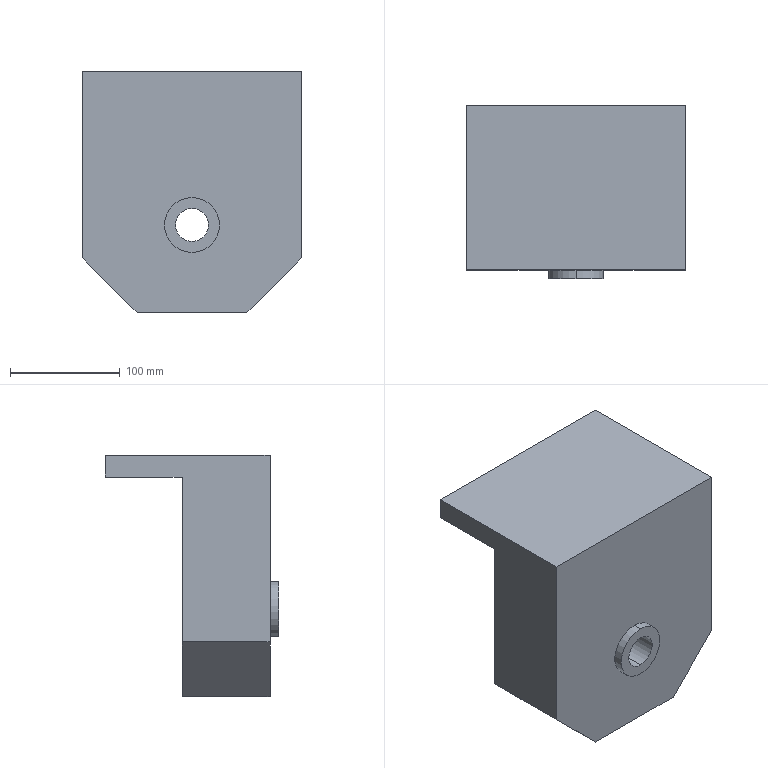Component | SolidWorks | HZ022-A001-D001-1 | 1 solid | 21 faces | box 200 x 158 x 220 mm | volume 3538459 mm3 | plane 13 | cylinder 8 | commonest cylinder face diameters 50 x4 16 x2 30 x2 | material AL6061
build123d program:
from build123d import *

# Parameters (mm, degrees)
SKETCH1_2_W               = 200
SKETCH1_2_H               = 220
BOSS_EXTRUDE1_DEPTH       = 150
SKETCH2_W                 = 200
SKETCH2_H                 = 200
CUT_EXTRUDE1_DEPTH        = 70
SKETCH3_R                 = 25
CUT_EXTRUDE2_DEPTH        = 5
SKETCH4_R                 = 25
BOSS_EXTRUDE2_DEPTH       = 8
SKETCH5_R                 = 15
CUT_EXTRUDE3_DEPTH        = 217.942
CHAMFER1_SIZE             = 50
SKETCH1_R                 = 8
MOTORSHAFTCLEARANCE_DEPTH = 26


with BuildPart() as part:
    # Sketch1_2 → Boss-Extrude1 (new body)
    with BuildSketch(Plane(origin=(0, 0, 0), x_dir=(1, 0, 0), z_dir=(0, 1, 0))):
        Rectangle(SKETCH1_2_W, SKETCH1_2_H)
    extrude(amount=BOSS_EXTRUDE1_DEPTH)

    # Sketch2 → Cut-Extrude1 (cut)
    with BuildSketch(Plane(origin=(0, 150, 0), x_dir=(1, 0, 0), z_dir=(0, 1, 0))):
        with Locations((0, 10)):
            Rectangle(SKETCH2_W, SKETCH2_H)
    extrude(amount=-CUT_EXTRUDE1_DEPTH, mode=Mode.SUBTRACT)

    # Sketch3 → Cut-Extrude2 (cut)
    with BuildSketch(Plane(origin=(0, 80, 0), x_dir=(1, 0, 0), z_dir=(0, 1, 0))):
        with Locations(Location((0, -50, 0), (0, 0, 270))):
            Circle(SKETCH3_R)
    extrude(amount=-CUT_EXTRUDE2_DEPTH, mode=Mode.SUBTRACT)

    # Sketch4 → Boss-Extrude2 (add)
    with BuildSketch(Plane.XZ):
        with Locations(Location((0, -30, 0), (0, 0, 90))):
            Circle(SKETCH4_R)
    extrude(amount=BOSS_EXTRUDE2_DEPTH)

    # Sketch5 → Cut-Extrude3 (cut, through all)
    with BuildSketch(Plane.XZ.offset(8)):
        with Locations(Location((0, -30, 0), (0, 0, 270))):
            Circle(SKETCH5_R)
    extrude(amount=-CUT_EXTRUDE3_DEPTH, mode=Mode.SUBTRACT)

    # Chamfer1
    chamfer1_edges = [part.edges().sort_by_distance(p)[0] for p in [
        (-100, 40, -110),
        (100, 40, -110),
    ]]
    chamfer(chamfer1_edges, length=CHAMFER1_SIZE)

    # Sketch1 → MotorShaftClearance (cut)
    with BuildSketch(Plane(origin=(0, 75, 0), x_dir=(1, 0, 0), z_dir=(0, 1, 0))):
        with Locations(Location((0, -50, 0), (0, 0, 270))):
            Circle(SKETCH1_R)
    extrude(amount=-MOTORSHAFTCLEARANCE_DEPTH, mode=Mode.SUBTRACT)


solid = part.part

# Placed as in the assembly
solid = solid.moved(Location((-12.865, -151.602, 510), (0, 0, 0)))
STEP:
#1=COLOUR_RGB('',0.7922,0.8196,0.9333);
#2=FILL_AREA_STYLE_COLOUR('',#1);
#3=FILL_AREA_STYLE('',(#2));
#4=SURFACE_STYLE_FILL_AREA(#3);
#5=SURFACE_SIDE_STYLE('',(#4));
#6=SURFACE_STYLE_USAGE(.BOTH.,#5);
#7=PRESENTATION_STYLE_ASSIGNMENT((#6));
#8=CARTESIAN_POINT('',(-0.5065,-4.039,21.732));
#9=VERTEX_POINT('',#8);
#10=CARTESIAN_POINT('',(-0.5065,-4.039,22.362));
#11=VERTEX_POINT('',#10);
#12=CARTESIAN_POINT('',(-0.5065,-4.039,22.047));
#13=DIRECTION('',(0.,1.,0.));
#14=DIRECTION('',(0.,0.,1.));
#15=AXIS2_PLACEMENT_3D('',#12,#13,#14);
#16=CIRCLE('',#15,0.315);
#17=EDGE_CURVE('',#9,#11,#16,.T.);
#18=ORIENTED_EDGE('',*,*,#17,.F.);
#19=CARTESIAN_POINT('',(-0.5065,-3.016,21.732));
#20=VERTEX_POINT('',#19);
#21=CARTESIAN_POINT('',(-0.5065,-4.039,21.732));
#22=DIRECTION('',(0.,1.,0.));
#23=VECTOR('',#22,39.37);
#24=LINE('',#21,#23);
#25=EDGE_CURVE('',#9,#20,#24,.T.);
#26=ORIENTED_EDGE('',*,*,#25,.T.);
#27=CARTESIAN_POINT('',(-0.5065,-3.016,22.362));
#28=VERTEX_POINT('',#27);
#29=CARTESIAN_POINT('',(-0.5065,-3.016,22.047));
#30=DIRECTION('',(0.,1.,0.));
#31=DIRECTION('',(0.,0.,1.));
#32=AXIS2_PLACEMENT_3D('',#29,#30,#31);
#33=CIRCLE('',#32,0.315);
#34=EDGE_CURVE('',#20,#28,#33,.T.);
#35=ORIENTED_EDGE('',*,*,#34,.T.);
#36=CARTESIAN_POINT('',(-0.5065,-4.039,22.362));
#37=DIRECTION('',(0.,1.,0.));
#38=VECTOR('',#37,39.37);
#39=LINE('',#36,#38);
#40=EDGE_CURVE('',#11,#28,#39,.T.);
#41=ORIENTED_EDGE('',*,*,#40,.F.);
#42=EDGE_LOOP('',(#18,#26,#35,#41));
#43=FACE_OUTER_BOUND('',#42,.T.);
#44=CARTESIAN_POINT('',(-0.5065,-4.039,22.047));
#45=DIRECTION('',(0.,1.,0.));
#46=DIRECTION('',(0.,0.,1.));
#47=AXIS2_PLACEMENT_3D('',#44,#45,#46);
#48=CYLINDRICAL_SURFACE('',#47,0.315);
#49=ADVANCED_FACE('',(#43),#48,.F.);
#50=CARTESIAN_POINT('',(-0.5065,-2.819,18.307));
#51=VERTEX_POINT('',#50);
#52=CARTESIAN_POINT('',(-0.5065,-2.819,19.488));
#53=VERTEX_POINT('',#52);
#54=CARTESIAN_POINT('',(-0.5065,-2.819,18.898));
#55=DIRECTION('',(0.,1.,0.));
#56=DIRECTION('',(0.,0.,1.));
#57=AXIS2_PLACEMENT_3D('',#54,#55,#56);
#58=CIRCLE('',#57,0.5906);
#59=EDGE_CURVE('',#51,#53,#58,.T.);
#60=ORIENTED_EDGE('',*,*,#59,.T.);
#61=CARTESIAN_POINT('',(-0.5065,-6.284,19.488));
#62=VERTEX_POINT('',#61);
#63=CARTESIAN_POINT('',(-0.5065,-0.06309,19.488));
#64=DIRECTION('',(0.,-1.,0.));
#65=VECTOR('',#64,39.37);
#66=LINE('',#63,#65);
#67=EDGE_CURVE('',#53,#62,#66,.T.);
#68=ORIENTED_EDGE('',*,*,#67,.T.);
#69=CARTESIAN_POINT('',(-0.5065,-6.284,18.307));
#70=VERTEX_POINT('',#69);
#71=CARTESIAN_POINT('',(-0.5065,-6.284,18.898));
#72=DIRECTION('',(0.,-1.,0.));
#73=DIRECTION('',(0.,0.,-1.));
#74=AXIS2_PLACEMENT_3D('',#71,#72,#73);
#75=CIRCLE('',#74,0.5906);
#76=EDGE_CURVE('',#62,#70,#75,.T.);
#77=ORIENTED_EDGE('',*,*,#76,.T.);
#78=CARTESIAN_POINT('',(-0.5065,-0.06309,18.307));
#79=DIRECTION('',(0.,-1.,0.));
#80=VECTOR('',#79,39.37);
#81=LINE('',#78,#80);
#82=EDGE_CURVE('',#51,#70,#81,.T.);
#83=ORIENTED_EDGE('',*,*,#82,.F.);
#84=EDGE_LOOP('',(#60,#68,#77,#83));
#85=FACE_OUTER_BOUND('',#84,.T.);
#86=CARTESIAN_POINT('',(-0.5065,-0.06309,18.898));
#87=DIRECTION('',(0.,-1.,0.));
#88=DIRECTION('',(0.,0.,-1.));
#89=AXIS2_PLACEMENT_3D('',#86,#87,#88);
#90=CYLINDRICAL_SURFACE('',#89,0.5906);
#91=ADVANCED_FACE('',(#85),#90,.F.);
#92=CARTESIAN_POINT('',(-0.5065,-6.284,17.913));
#93=VERTEX_POINT('',#92);
#94=CARTESIAN_POINT('',(-0.5065,-6.284,19.882));
#95=VERTEX_POINT('',#94);
#96=CARTESIAN_POINT('',(-0.5065,-6.284,18.898));
#97=DIRECTION('',(0.,-1.,0.));
#98=DIRECTION('',(0.,0.,-1.));
#99=AXIS2_PLACEMENT_3D('',#96,#97,#98);
#100=CIRCLE('',#99,0.9843);
#101=EDGE_CURVE('',#93,#95,#100,.T.);
#102=ORIENTED_EDGE('',*,*,#101,.F.);
#103=CARTESIAN_POINT('',(-0.5065,-5.969,17.913));
#104=VERTEX_POINT('',#103);
#105=CARTESIAN_POINT('',(-0.5065,-6.284,17.913));
#106=DIRECTION('',(0.,1.,0.));
#107=VECTOR('',#106,39.37);
#108=LINE('',#105,#107);
#109=EDGE_CURVE('',#93,#104,#108,.T.);
#110=ORIENTED_EDGE('',*,*,#109,.T.);
#111=CARTESIAN_POINT('',(-0.5065,-5.969,19.882));
#112=VERTEX_POINT('',#111);
#113=CARTESIAN_POINT('',(-0.5065,-5.969,18.898));
#114=DIRECTION('',(0.,-1.,0.));
#115=DIRECTION('',(0.,0.,1.));
#116=AXIS2_PLACEMENT_3D('',#113,#114,#115);
#117=CIRCLE('',#116,0.9843);
#118=EDGE_CURVE('',#104,#112,#117,.T.);
#119=ORIENTED_EDGE('',*,*,#118,.T.);
#120=CARTESIAN_POINT('',(-0.5065,-6.284,19.882));
#121=DIRECTION('',(0.,1.,0.));
#122=VECTOR('',#121,39.37);
#123=LINE('',#120,#122);
#124=EDGE_CURVE('',#95,#112,#123,.T.);
#125=ORIENTED_EDGE('',*,*,#124,.F.);
#126=EDGE_LOOP('',(#102,#110,#119,#125));
#127=FACE_OUTER_BOUND('',#126,.T.);
#128=CARTESIAN_POINT('',(-0.5065,-6.284,18.898));
#129=DIRECTION('',(0.,1.,0.));
#130=DIRECTION('',(0.,0.,1.));
#131=AXIS2_PLACEMENT_3D('',#128,#129,#130);
#132=CYLINDRICAL_SURFACE('',#131,0.9843);
#133=ADVANCED_FACE('',(#127),#132,.T.);
#134=CARTESIAN_POINT('',(-0.5065,-3.016,21.063));
#135=VERTEX_POINT('',#134);
#136=CARTESIAN_POINT('',(-0.5065,-3.016,23.031));
#137=VERTEX_POINT('',#136);
#138=CARTESIAN_POINT('',(-0.5065,-3.016,22.047));
#139=DIRECTION('',(0.,1.,0.));
#140=DIRECTION('',(0.,0.,1.));
#141=AXIS2_PLACEMENT_3D('',#138,#139,#140);
#142=CIRCLE('',#141,0.9843);
#143=EDGE_CURVE('',#135,#137,#142,.T.);
#144=ORIENTED_EDGE('',*,*,#143,.F.);
#145=CARTESIAN_POINT('',(-0.5065,-2.819,21.063));
#146=VERTEX_POINT('',#145);
#147=CARTESIAN_POINT('',(-0.5065,-3.016,21.063));
#148=DIRECTION('',(0.,1.,0.));
#149=VECTOR('',#148,39.37);
#150=LINE('',#147,#149);
#151=EDGE_CURVE('',#135,#146,#150,.T.);
#152=ORIENTED_EDGE('',*,*,#151,.T.);
#153=CARTESIAN_POINT('',(-0.5065,-2.819,23.031));
#154=VERTEX_POINT('',#153);
#155=CARTESIAN_POINT('',(-0.5065,-2.819,22.047));
#156=DIRECTION('',(0.,1.,0.));
#157=DIRECTION('',(0.,0.,1.));
#158=AXIS2_PLACEMENT_3D('',#155,#156,#157);
#159=CIRCLE('',#158,0.9843);
#160=EDGE_CURVE('',#146,#154,#159,.T.);
#161=ORIENTED_EDGE('',*,*,#160,.T.);
#162=CARTESIAN_POINT('',(-0.5065,-3.016,23.031));
#163=DIRECTION('',(0.,1.,0.));
#164=VECTOR('',#163,39.37);
#165=LINE('',#162,#164);
#166=EDGE_CURVE('',#137,#154,#165,.T.);
#167=ORIENTED_EDGE('',*,*,#166,.F.);
#168=EDGE_LOOP('',(#144,#152,#161,#167));
#169=FACE_OUTER_BOUND('',#168,.T.);
#170=CARTESIAN_POINT('',(-0.5065,-3.016,22.047));
#171=DIRECTION('',(0.,1.,0.));
#172=DIRECTION('',(0.,0.,1.));
#173=AXIS2_PLACEMENT_3D('',#170,#171,#172);
#174=CYLINDRICAL_SURFACE('',#173,0.9843);
#175=ADVANCED_FACE('',(#169),#174,.F.);
#176=CARTESIAN_POINT('',(1.462,-2.819,15.748));
#177=VERTEX_POINT('',#176);
#178=CARTESIAN_POINT('',(-2.475,-2.819,15.748));
#179=VERTEX_POINT('',#178);
#180=CARTESIAN_POINT('',(3.431,-2.819,15.748));
#181=DIRECTION('',(-1.,0.,-0.));
#182=VECTOR('',#181,39.37);
#183=LINE('',#180,#182);
#184=EDGE_CURVE('',#177,#179,#183,.T.);
#185=ORIENTED_EDGE('',*,*,#184,.F.);
#186=CARTESIAN_POINT('',(1.462,-5.969,15.748));
#187=VERTEX_POINT('',#186);
#188=CARTESIAN_POINT('',(1.462,-0.06309,15.748));
#189=DIRECTION('',(0.,-1.,0.));
#190=VECTOR('',#189,39.37);
#191=LINE('',#188,#190);
#192=EDGE_CURVE('',#177,#187,#191,.T.);
#193=ORIENTED_EDGE('',*,*,#192,.T.);
#194=CARTESIAN_POINT('',(-2.475,-5.969,15.748));
#195=VERTEX_POINT('',#194);
#196=CARTESIAN_POINT('',(-0.5065,-5.969,15.748));
#197=DIRECTION('',(1.,0.,0.));
#198=VECTOR('',#197,39.37);
#199=LINE('',#196,#198);
#200=EDGE_CURVE('',#195,#187,#199,.T.);
#201=ORIENTED_EDGE('',*,*,#200,.F.);
#202=CARTESIAN_POINT('',(-2.475,-2.819,15.748));
#203=DIRECTION('',(0.,1.,0.));
#204=VECTOR('',#203,39.37);
#205=LINE('',#202,#204);
#206=EDGE_CURVE('',#195,#179,#205,.T.);
#207=ORIENTED_EDGE('',*,*,#206,.T.);
#208=EDGE_LOOP('',(#185,#193,#201,#207));
#209=FACE_OUTER_BOUND('',#208,.T.);
#210=CARTESIAN_POINT('',(-0.5065,-0.06309,15.748));
#211=DIRECTION('',(0.,0.,-1.));
#212=DIRECTION('',(-1.,0.,-0.));
#213=AXIS2_PLACEMENT_3D('',#210,#211,#212);
#214=PLANE('',#213);
#215=ADVANCED_FACE('',(#209),#214,.T.);
#216=CARTESIAN_POINT('',(3.431,-5.969,17.717));
#217=VERTEX_POINT('',#216);
#218=CARTESIAN_POINT('',(3.431,-5.969,24.409));
#219=VERTEX_POINT('',#218);
#220=CARTESIAN_POINT('',(3.431,-5.969,20.079));
#221=DIRECTION('',(0.,0.,1.));
#222=VECTOR('',#221,39.37);
#223=LINE('',#220,#222);
#224=EDGE_CURVE('',#217,#219,#223,.T.);
#225=ORIENTED_EDGE('',*,*,#224,.F.);
#226=CARTESIAN_POINT('',(3.431,-2.819,17.717));
#227=VERTEX_POINT('',#226);
#228=CARTESIAN_POINT('',(3.431,-0.06309,17.717));
#229=DIRECTION('',(0.,1.,0.));
#230=VECTOR('',#229,39.37);
#231=LINE('',#228,#230);
#232=EDGE_CURVE('',#217,#227,#231,.T.);
#233=ORIENTED_EDGE('',*,*,#232,.T.);
#234=CARTESIAN_POINT('',(3.431,-2.819,23.622));
#235=VERTEX_POINT('',#234);
#236=CARTESIAN_POINT('',(3.431,-2.819,23.622));
#237=DIRECTION('',(0.,0.,-1.));
#238=VECTOR('',#237,39.37);
#239=LINE('',#236,#238);
#240=EDGE_CURVE('',#235,#227,#239,.T.);
#241=ORIENTED_EDGE('',*,*,#240,.F.);
#242=CARTESIAN_POINT('',(3.431,-0.06309,23.622));
#243=VERTEX_POINT('',#242);
#244=CARTESIAN_POINT('',(3.431,-2.819,23.622));
#245=DIRECTION('',(0.,1.,0.));
#246=VECTOR('',#245,39.37);
#247=LINE('',#244,#246);
#248=EDGE_CURVE('',#235,#243,#247,.T.);
#249=ORIENTED_EDGE('',*,*,#248,.T.);
#250=CARTESIAN_POINT('',(3.431,-0.06309,24.409));
#251=VERTEX_POINT('',#250);
#252=CARTESIAN_POINT('',(3.431,-0.06309,20.079));
#253=DIRECTION('',(0.,0.,1.));
#254=VECTOR('',#253,39.37);
#255=LINE('',#252,#254);
#256=EDGE_CURVE('',#243,#251,#255,.T.);
#257=ORIENTED_EDGE('',*,*,#256,.T.);
#258=CARTESIAN_POINT('',(3.431,-0.06309,24.409));
#259=DIRECTION('',(0.,-1.,0.));
#260=VECTOR('',#259,39.37);
#261=LINE('',#258,#260);
#262=EDGE_CURVE('',#251,#219,#261,.T.);
#263=ORIENTED_EDGE('',*,*,#262,.T.);
#264=EDGE_LOOP('',(#225,#233,#241,#249,#257,#263));
#265=FACE_OUTER_BOUND('',#264,.T.);
#266=CARTESIAN_POINT('',(3.431,-0.06309,20.079));
#267=DIRECTION('',(1.,0.,-0.));
#268=DIRECTION('',(-0.,0.,-1.));
#269=AXIS2_PLACEMENT_3D('',#266,#267,#268);
#270=PLANE('',#269);
#271=ADVANCED_FACE('',(#265),#270,.T.);
#272=CARTESIAN_POINT('',(-4.444,-2.819,17.717));
#273=VERTEX_POINT('',#272);
#274=CARTESIAN_POINT('',(-4.444,-2.819,23.622));
#275=VERTEX_POINT('',#274);
#276=CARTESIAN_POINT('',(-4.444,-2.819,23.622));
#277=DIRECTION('',(0.,0.,1.));
#278=VECTOR('',#277,39.37);
#279=LINE('',#276,#278);
#280=EDGE_CURVE('',#273,#275,#279,.T.);
#281=ORIENTED_EDGE('',*,*,#280,.F.);
#282=CARTESIAN_POINT('',(-4.444,-5.969,17.717));
#283=VERTEX_POINT('',#282);
#284=CARTESIAN_POINT('',(-4.444,-5.969,17.717));
#285=DIRECTION('',(0.,-1.,0.));
#286=VECTOR('',#285,39.37);
#287=LINE('',#284,#286);
#288=EDGE_CURVE('',#273,#283,#287,.T.);
#289=ORIENTED_EDGE('',*,*,#288,.T.);
#290=CARTESIAN_POINT('',(-4.444,-5.969,24.409));
#291=VERTEX_POINT('',#290);
#292=CARTESIAN_POINT('',(-4.444,-5.969,20.079));
#293=DIRECTION('',(0.,0.,1.));
#294=VECTOR('',#293,39.37);
#295=LINE('',#292,#294);
#296=EDGE_CURVE('',#283,#291,#295,.T.);
#297=ORIENTED_EDGE('',*,*,#296,.T.);
#298=CARTESIAN_POINT('',(-4.444,-0.06309,24.409));
#299=VERTEX_POINT('',#298);
#300=CARTESIAN_POINT('',(-4.444,-0.06309,24.409));
#301=DIRECTION('',(0.,-1.,0.));
#302=VECTOR('',#301,39.37);
#303=LINE('',#300,#302);
#304=EDGE_CURVE('',#299,#291,#303,.T.);
#305=ORIENTED_EDGE('',*,*,#304,.F.);
#306=CARTESIAN_POINT('',(-4.444,-0.06309,23.622));
#307=VERTEX_POINT('',#306);
#308=CARTESIAN_POINT('',(-4.444,-0.06309,20.079));
#309=DIRECTION('',(0.,0.,1.));
#310=VECTOR('',#309,39.37);
#311=LINE('',#308,#310);
#312=EDGE_CURVE('',#307,#299,#311,.T.);
#313=ORIENTED_EDGE('',*,*,#312,.F.);
#314=CARTESIAN_POINT('',(-4.444,-2.819,23.622));
#315=DIRECTION('',(0.,1.,0.));
#316=VECTOR('',#315,39.37);
#317=LINE('',#314,#316);
#318=EDGE_CURVE('',#275,#307,#317,.T.);
#319=ORIENTED_EDGE('',*,*,#318,.F.);
#320=EDGE_LOOP('',(#281,#289,#297,#305,#313,#319));
#321=FACE_OUTER_BOUND('',#320,.T.);
#322=CARTESIAN_POINT('',(-4.444,-0.06309,20.079));
#323=DIRECTION('',(1.,0.,-0.));
#324=DIRECTION('',(-0.,0.,-1.));
#325=AXIS2_PLACEMENT_3D('',#322,#323,#324);
#326=PLANE('',#325);
#327=ADVANCED_FACE('',(#321),#326,.F.);
#328=CARTESIAN_POINT('',(-0.5065,-5.969,24.409));
#329=DIRECTION('',(1.,0.,0.));
#330=VECTOR('',#329,39.37);
#331=LINE('',#328,#330);
#332=EDGE_CURVE('',#291,#219,#331,.T.);
#333=ORIENTED_EDGE('',*,*,#332,.T.);
#334=ORIENTED_EDGE('',*,*,#262,.F.);
#335=CARTESIAN_POINT('',(-0.5065,-0.06309,24.409));
#336=DIRECTION('',(1.,0.,0.));
#337=VECTOR('',#336,39.37);
#338=LINE('',#335,#337);
#339=EDGE_CURVE('',#299,#251,#338,.T.);
#340=ORIENTED_EDGE('',*,*,#339,.F.);
#341=ORIENTED_EDGE('',*,*,#304,.T.);
#342=EDGE_LOOP('',(#333,#334,#340,#341));
#343=FACE_OUTER_BOUND('',#342,.T.);
#344=CARTESIAN_POINT('',(-0.5065,-0.06309,24.409));
#345=DIRECTION('',(0.,0.,-1.));
#346=DIRECTION('',(-1.,0.,0.));
#347=AXIS2_PLACEMENT_3D('',#344,#345,#346);
#348=PLANE('',#347);
#349=ADVANCED_FACE('',(#343),#348,.F.);
#350=CARTESIAN_POINT('',(3.431,-0.06309,23.622));
#351=DIRECTION('',(1.,0.,0.));
#352=VECTOR('',#351,39.37);
#353=LINE('',#350,#352);
#354=EDGE_CURVE('',#307,#243,#353,.T.);
#355=ORIENTED_EDGE('',*,*,#354,.F.);
#356=ORIENTED_EDGE('',*,*,#312,.T.);
#357=ORIENTED_EDGE('',*,*,#339,.T.);
#358=ORIENTED_EDGE('',*,*,#256,.F.);
#359=EDGE_LOOP('',(#355,#356,#357,#358));
#360=FACE_OUTER_BOUND('',#359,.T.);
#361=CARTESIAN_POINT('',(-0.5065,-0.06309,20.079));
#362=DIRECTION('',(0.,1.,0.));
#363=DIRECTION('',(0.,0.,1.));
#364=AXIS2_PLACEMENT_3D('',#361,#362,#363);
#365=PLANE('',#364);
#366=ADVANCED_FACE('',(#360),#365,.T.);
#367=CARTESIAN_POINT('',(-0.5065,-5.969,18.898));
#368=DIRECTION('',(0.,-1.,0.));
#369=DIRECTION('',(0.,0.,1.));
#370=AXIS2_PLACEMENT_3D('',#367,#368,#369);
#371=CIRCLE('',#370,0.9843);
#372=EDGE_CURVE('',#112,#104,#371,.T.);
#373=ORIENTED_EDGE('',*,*,#372,.F.);
#374=ORIENTED_EDGE('',*,*,#118,.F.);
#375=EDGE_LOOP('',(#373,#374));
#376=FACE_BOUND('',#375,.T.);
#377=ORIENTED_EDGE('',*,*,#200,.T.);
#378=CARTESIAN_POINT('',(1.462,-5.969,15.748));
#379=DIRECTION('',(0.7071,0.,0.7071));
#380=VECTOR('',#379,39.37);
#381=LINE('',#378,#380);
#382=EDGE_CURVE('',#187,#217,#381,.T.);
#383=ORIENTED_EDGE('',*,*,#382,.T.);
#384=ORIENTED_EDGE('',*,*,#224,.T.);
#385=ORIENTED_EDGE('',*,*,#332,.F.);
#386=ORIENTED_EDGE('',*,*,#296,.F.);
#387=CARTESIAN_POINT('',(-4.444,-5.969,17.717));
#388=DIRECTION('',(0.7071,0.,-0.7071));
#389=VECTOR('',#388,39.37);
#390=LINE('',#387,#389);
#391=EDGE_CURVE('',#283,#195,#390,.T.);
#392=ORIENTED_EDGE('',*,*,#391,.T.);
#393=EDGE_LOOP('',(#377,#383,#384,#385,#386,#392));
#394=FACE_OUTER_BOUND('',#393,.T.);
#395=CARTESIAN_POINT('',(-0.5065,-5.969,20.079));
#396=DIRECTION('',(0.,1.,0.));
#397=DIRECTION('',(0.,0.,1.));
#398=AXIS2_PLACEMENT_3D('',#395,#396,#397);
#399=PLANE('',#398);
#400=ADVANCED_FACE('',(#376,#394),#399,.F.);
#401=ORIENTED_EDGE('',*,*,#354,.T.);
#402=ORIENTED_EDGE('',*,*,#248,.F.);
#403=CARTESIAN_POINT('',(3.431,-2.819,23.622));
#404=DIRECTION('',(1.,0.,0.));
#405=VECTOR('',#404,39.37);
#406=LINE('',#403,#405);
#407=EDGE_CURVE('',#275,#235,#406,.T.);
#408=ORIENTED_EDGE('',*,*,#407,.F.);
#409=ORIENTED_EDGE('',*,*,#318,.T.);
#410=EDGE_LOOP('',(#401,#402,#408,#409));
#411=FACE_OUTER_BOUND('',#410,.T.);
#412=CARTESIAN_POINT('',(3.431,-2.819,23.622));
#413=DIRECTION('',(0.,0.,1.));
#414=DIRECTION('',(1.,0.,0.));
#415=AXIS2_PLACEMENT_3D('',#412,#413,#414);
#416=PLANE('',#415);
#417=ADVANCED_FACE('',(#411),#416,.F.);
#418=ORIENTED_EDGE('',*,*,#59,.F.);
#419=CARTESIAN_POINT('',(-0.5065,-2.819,18.898));
#420=DIRECTION('',(0.,1.,0.));
#421=DIRECTION('',(0.,0.,1.));
#422=AXIS2_PLACEMENT_3D('',#419,#420,#421);
#423=CIRCLE('',#422,0.5906);
#424=EDGE_CURVE('',#53,#51,#423,.T.);
#425=ORIENTED_EDGE('',*,*,#424,.F.);
#426=EDGE_LOOP('',(#418,#425));
#427=FACE_BOUND('',#426,.T.);
#428=CARTESIAN_POINT('',(-0.5065,-2.819,22.047));
#429=DIRECTION('',(0.,1.,0.));
#430=DIRECTION('',(0.,0.,1.));
#431=AXIS2_PLACEMENT_3D('',#428,#429,#430);
#432=CIRCLE('',#431,0.9843);
#433=EDGE_CURVE('',#154,#146,#432,.T.);
#434=ORIENTED_EDGE('',*,*,#433,.F.);
#435=ORIENTED_EDGE('',*,*,#160,.F.);
#436=EDGE_LOOP('',(#434,#435));
#437=FACE_BOUND('',#436,.T.);
#438=ORIENTED_EDGE('',*,*,#240,.T.);
#439=CARTESIAN_POINT('',(2.643,-2.819,16.929));
#440=DIRECTION('',(-0.7071,0.,-0.7071));
#441=VECTOR('',#440,39.37);
#442=LINE('',#439,#441);
#443=EDGE_CURVE('',#227,#177,#442,.T.);
#444=ORIENTED_EDGE('',*,*,#443,.T.);
#445=ORIENTED_EDGE('',*,*,#184,.T.);
#446=CARTESIAN_POINT('',(-3.656,-2.819,16.929));
#447=DIRECTION('',(-0.7071,0.,0.7071));
#448=VECTOR('',#447,39.37);
#449=LINE('',#446,#448);
#450=EDGE_CURVE('',#179,#273,#449,.T.);
#451=ORIENTED_EDGE('',*,*,#450,.T.);
#452=ORIENTED_EDGE('',*,*,#280,.T.);
#453=ORIENTED_EDGE('',*,*,#407,.T.);
#454=EDGE_LOOP('',(#438,#444,#445,#451,#452,#453));
#455=FACE_OUTER_BOUND('',#454,.T.);
#456=CARTESIAN_POINT('',(-0.5065,-2.819,20.079));
#457=DIRECTION('',(0.,1.,0.));
#458=DIRECTION('',(0.,0.,1.));
#459=AXIS2_PLACEMENT_3D('',#456,#457,#458);
#460=PLANE('',#459);
#461=ADVANCED_FACE('',(#427,#437,#455),#460,.T.);
#462=ORIENTED_EDGE('',*,*,#151,.F.);
#463=CARTESIAN_POINT('',(-0.5065,-3.016,22.047));
#464=DIRECTION('',(0.,1.,0.));
#465=DIRECTION('',(0.,0.,1.));
#466=AXIS2_PLACEMENT_3D('',#463,#464,#465);
#467=CIRCLE('',#466,0.9843);
#468=EDGE_CURVE('',#137,#135,#467,.T.);
#469=ORIENTED_EDGE('',*,*,#468,.F.);
#470=ORIENTED_EDGE('',*,*,#166,.T.);
#471=ORIENTED_EDGE('',*,*,#433,.T.);
#472=EDGE_LOOP('',(#462,#469,#470,#471));
#473=FACE_OUTER_BOUND('',#472,.T.);
#474=CARTESIAN_POINT('',(-0.5065,-3.016,22.047));
#475=DIRECTION('',(0.,1.,0.));
#476=DIRECTION('',(0.,0.,1.));
#477=AXIS2_PLACEMENT_3D('',#474,#475,#476);
#478=CYLINDRICAL_SURFACE('',#477,0.9843);
#479=ADVANCED_FACE('',(#473),#478,.F.);
#480=CARTESIAN_POINT('',(-0.5065,-3.016,22.047));
#481=DIRECTION('',(0.,1.,0.));
#482=DIRECTION('',(0.,0.,1.));
#483=AXIS2_PLACEMENT_3D('',#480,#481,#482);
#484=CIRCLE('',#483,0.315);
#485=EDGE_CURVE('',#28,#20,#484,.T.);
#486=ORIENTED_EDGE('',*,*,#485,.F.);
#487=ORIENTED_EDGE('',*,*,#34,.F.);
#488=EDGE_LOOP('',(#486,#487));
#489=FACE_BOUND('',#488,.T.);
#490=ORIENTED_EDGE('',*,*,#468,.T.);
#491=ORIENTED_EDGE('',*,*,#143,.T.);
#492=EDGE_LOOP('',(#490,#491));
#493=FACE_OUTER_BOUND('',#492,.T.);
#494=CARTESIAN_POINT('',(-0.5065,-3.016,22.047));
#495=DIRECTION('',(0.,1.,0.));
#496=DIRECTION('',(0.,0.,1.));
#497=AXIS2_PLACEMENT_3D('',#494,#495,#496);
#498=PLANE('',#497);
#499=ADVANCED_FACE('',(#489,#493),#498,.T.);
#500=ORIENTED_EDGE('',*,*,#109,.F.);
#501=CARTESIAN_POINT('',(-0.5065,-6.284,18.898));
#502=DIRECTION('',(0.,-1.,0.));
#503=DIRECTION('',(0.,0.,-1.));
#504=AXIS2_PLACEMENT_3D('',#501,#502,#503);
#505=CIRCLE('',#504,0.9843);
#506=EDGE_CURVE('',#95,#93,#505,.T.);
#507=ORIENTED_EDGE('',*,*,#506,.F.);
#508=ORIENTED_EDGE('',*,*,#124,.T.);
#509=ORIENTED_EDGE('',*,*,#372,.T.);
#510=EDGE_LOOP('',(#500,#507,#508,#509));
#511=FACE_OUTER_BOUND('',#510,.T.);
#512=CARTESIAN_POINT('',(-0.5065,-6.284,18.898));
#513=DIRECTION('',(0.,1.,0.));
#514=DIRECTION('',(0.,0.,1.));
#515=AXIS2_PLACEMENT_3D('',#512,#513,#514);
#516=CYLINDRICAL_SURFACE('',#515,0.9843);
#517=ADVANCED_FACE('',(#511),#516,.T.);
#518=CARTESIAN_POINT('',(-0.5065,-6.284,18.898));
#519=DIRECTION('',(0.,-1.,0.));
#520=DIRECTION('',(0.,0.,-1.));
#521=AXIS2_PLACEMENT_3D('',#518,#519,#520);
#522=CIRCLE('',#521,0.5906);
#523=EDGE_CURVE('',#70,#62,#522,.T.);
#524=ORIENTED_EDGE('',*,*,#523,.F.);
#525=ORIENTED_EDGE('',*,*,#76,.F.);
#526=EDGE_LOOP('',(#524,#525));
#527=FACE_BOUND('',#526,.T.);
#528=ORIENTED_EDGE('',*,*,#506,.T.);
#529=ORIENTED_EDGE('',*,*,#101,.T.);
#530=EDGE_LOOP('',(#528,#529));
#531=FACE_OUTER_BOUND('',#530,.T.);
#532=CARTESIAN_POINT('',(-0.5065,-6.284,18.898));
#533=DIRECTION('',(0.,-1.,0.));
#534=DIRECTION('',(0.,0.,-1.));
#535=AXIS2_PLACEMENT_3D('',#532,#533,#534);
#536=PLANE('',#535);
#537=ADVANCED_FACE('',(#527,#531),#536,.T.);
#538=ORIENTED_EDGE('',*,*,#67,.F.);
#539=ORIENTED_EDGE('',*,*,#424,.T.);
#540=ORIENTED_EDGE('',*,*,#82,.T.);
#541=ORIENTED_EDGE('',*,*,#523,.T.);
#542=EDGE_LOOP('',(#538,#539,#540,#541));
#543=FACE_OUTER_BOUND('',#542,.T.);
#544=CARTESIAN_POINT('',(-0.5065,-0.06309,18.898));
#545=DIRECTION('',(0.,-1.,0.));
#546=DIRECTION('',(0.,0.,-1.));
#547=AXIS2_PLACEMENT_3D('',#544,#545,#546);
#548=CYLINDRICAL_SURFACE('',#547,0.5906);
#549=ADVANCED_FACE('',(#543),#548,.F.);
#550=ORIENTED_EDGE('',*,*,#443,.F.);
#551=ORIENTED_EDGE('',*,*,#232,.F.);
#552=ORIENTED_EDGE('',*,*,#382,.F.);
#553=ORIENTED_EDGE('',*,*,#192,.F.);
#554=EDGE_LOOP('',(#550,#551,#552,#553));
#555=FACE_OUTER_BOUND('',#554,.T.);
#556=CARTESIAN_POINT('',(1.462,-0.06309,15.748));
#557=DIRECTION('',(-0.7071,0.,0.7071));
#558=DIRECTION('',(0.,-1.,0.));
#559=AXIS2_PLACEMENT_3D('',#556,#557,#558);
#560=PLANE('',#559);
#561=ADVANCED_FACE('',(#555),#560,.F.);
#562=ORIENTED_EDGE('',*,*,#450,.F.);
#563=ORIENTED_EDGE('',*,*,#206,.F.);
#564=ORIENTED_EDGE('',*,*,#391,.F.);
#565=ORIENTED_EDGE('',*,*,#288,.F.);
#566=EDGE_LOOP('',(#562,#563,#564,#565));
#567=FACE_OUTER_BOUND('',#566,.T.);
#568=CARTESIAN_POINT('',(-4.444,-0.06309,17.717));
#569=DIRECTION('',(-0.7071,0.,-0.7071));
#570=DIRECTION('',(0.,1.,0.));
#571=AXIS2_PLACEMENT_3D('',#568,#569,#570);
#572=PLANE('',#571);
#573=ADVANCED_FACE('',(#567),#572,.T.);
#574=ORIENTED_EDGE('',*,*,#25,.F.);
#575=CARTESIAN_POINT('',(-0.5065,-4.039,22.047));
#576=DIRECTION('',(0.,1.,0.));
#577=DIRECTION('',(0.,0.,1.));
#578=AXIS2_PLACEMENT_3D('',#575,#576,#577);
#579=CIRCLE('',#578,0.315);
#580=EDGE_CURVE('',#11,#9,#579,.T.);
#581=ORIENTED_EDGE('',*,*,#580,.F.);
#582=ORIENTED_EDGE('',*,*,#40,.T.);
#583=ORIENTED_EDGE('',*,*,#485,.T.);
#584=EDGE_LOOP('',(#574,#581,#582,#583));
#585=FACE_OUTER_BOUND('',#584,.T.);
#586=CARTESIAN_POINT('',(-0.5065,-4.039,22.047));
#587=DIRECTION('',(0.,1.,0.));
#588=DIRECTION('',(0.,0.,1.));
#589=AXIS2_PLACEMENT_3D('',#586,#587,#588);
#590=CYLINDRICAL_SURFACE('',#589,0.315);
#591=ADVANCED_FACE('',(#585),#590,.F.);
#592=ORIENTED_EDGE('',*,*,#580,.T.);
#593=ORIENTED_EDGE('',*,*,#17,.T.);
#594=EDGE_LOOP('',(#592,#593));
#595=FACE_OUTER_BOUND('',#594,.T.);
#596=CARTESIAN_POINT('',(-0.5065,-4.039,22.047));
#597=DIRECTION('',(0.,1.,0.));
#598=DIRECTION('',(0.,0.,1.));
#599=AXIS2_PLACEMENT_3D('',#596,#597,#598);
#600=PLANE('',#599);
#601=ADVANCED_FACE('',(#595),#600,.T.);
#602=CLOSED_SHELL('',(#49,#91,#133,#175,#215,#271,#327,#349,#366,#400,#417,#461,#479,#499,#517,#537,#549,#561,#573,#591,#601));
#603=MANIFOLD_SOLID_BREP('',#602);
#604=STYLED_ITEM('',(#7),#603);
#605=PRESENTATION_LAYER_ASSIGNMENT('','',(#604));
#606=CARTESIAN_POINT('',(0.,0.,0.));
#607=DIRECTION('',(0.,0.,1.));
#608=DIRECTION('',(1.,0.,0.));
#609=AXIS2_PLACEMENT_3D('',#606,#607,#608);
#610=(LENGTH_UNIT()NAMED_UNIT(*)SI_UNIT($,.METRE.));
#611=LENGTH_MEASURE_WITH_UNIT(LENGTH_MEASURE(0.0254),#610);
#612=DIMENSIONAL_EXPONENTS(1.,0.,0.,0.,0.,0.,0.);
#613=(CONVERSION_BASED_UNIT('',#611)LENGTH_UNIT()NAMED_UNIT(#612));
#614=UNCERTAINTY_MEASURE_WITH_UNIT(LENGTH_MEASURE(0.00001),#613,'','');
#615=(NAMED_UNIT(*)PLANE_ANGLE_UNIT()SI_UNIT($,.RADIAN.));
#616=(NAMED_UNIT(*)SI_UNIT($,.STERADIAN.)SOLID_ANGLE_UNIT());
#617=(GEOMETRIC_REPRESENTATION_CONTEXT(3)GLOBAL_UNCERTAINTY_ASSIGNED_CONTEXT((#614))GLOBAL_UNIT_ASSIGNED_CONTEXT((#613,#615,#616))REPRESENTATION_CONTEXT('',''));
#618=ADVANCED_BREP_SHAPE_REPRESENTATION('',(#603,#609),#617);
#619=(LENGTH_UNIT()NAMED_UNIT(*)SI_UNIT($,.METRE.));
#620=LENGTH_MEASURE_WITH_UNIT(LENGTH_MEASURE(0.0254),#619);
#621=DIMENSIONAL_EXPONENTS(1.,0.,0.,0.,0.,0.,0.);
#622=(CONVERSION_BASED_UNIT('',#620)LENGTH_UNIT()NAMED_UNIT(#621));
#623=UNCERTAINTY_MEASURE_WITH_UNIT(LENGTH_MEASURE(0.00001),#622,'','');
#624=(NAMED_UNIT(*)PLANE_ANGLE_UNIT()SI_UNIT($,.RADIAN.));
#625=(NAMED_UNIT(*)SI_UNIT($,.STERADIAN.)SOLID_ANGLE_UNIT());
#626=(GEOMETRIC_REPRESENTATION_CONTEXT(3)GLOBAL_UNCERTAINTY_ASSIGNED_CONTEXT((#623))GLOBAL_UNIT_ASSIGNED_CONTEXT((#622,#624,#625))REPRESENTATION_CONTEXT('',''));
#627=MECHANICAL_DESIGN_GEOMETRIC_PRESENTATION_REPRESENTATION('',(#604),#626);